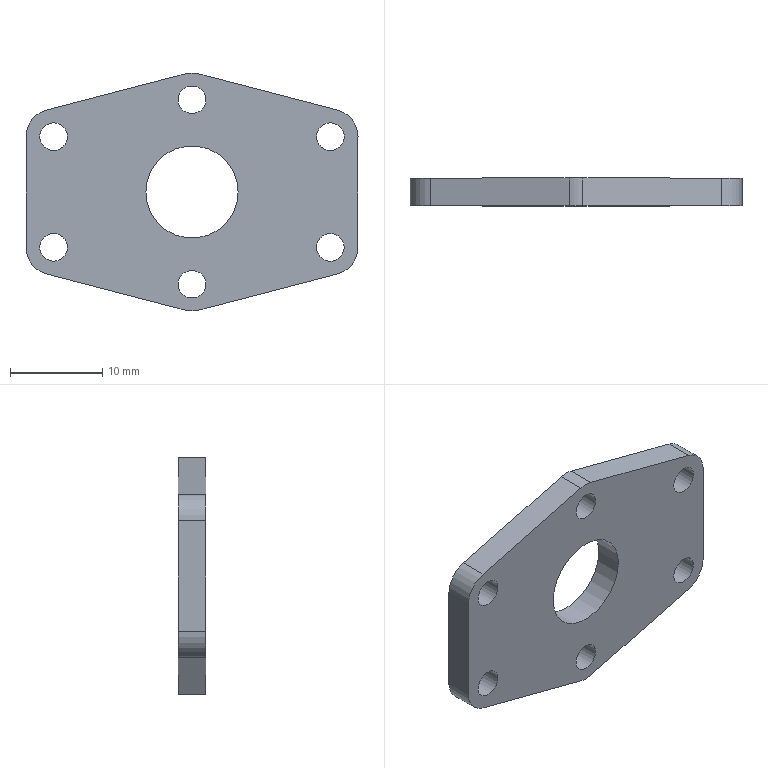Component | NX | 05E__27_2 | 1 solid | 21 faces | volume 1925 mm3 | cylinder 13 | plane 8 | commonest cylinder face diameters 6 x6 3 x6 10 x1